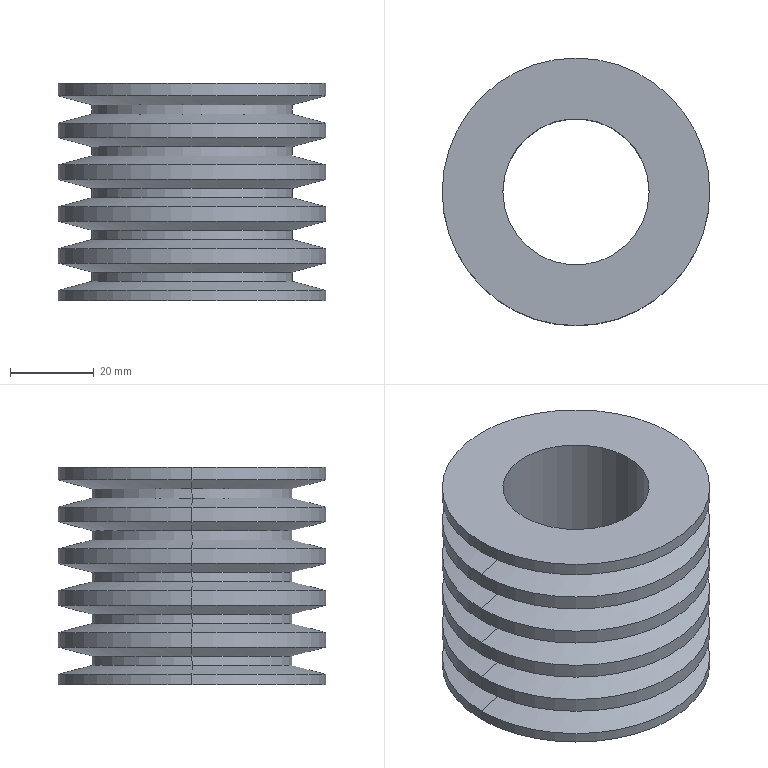Component | SolidWorks | SmallPulley-1 | 1 solid | 46 faces | box 64 x 64 x 52 mm | volume 85635 mm3 | cylinder 24 | cone 20 | plane 2 | commonest cylinder face diameters 64 x12 48 x10 35 x2
build123d program:
from build123d import *


with BuildPart() as part:
    # Sketch1 → Revolve1 (revolve)
    with BuildSketch(Plane(origin=(0, 0, 0), x_dir=(0, 0, -1), z_dir=(1, 0, 0)), mode=Mode.PRIVATE) as revolve1_sk:
        Polygon((49.535, 0), (52, 0), (52, -14.5), (0, -14.5), (0, 0), (3, 0), (5.144, -8), (7.391, -8), (9.535, 0), (13, 0), (15.144, -8), (17.391, -8), (19.535, 0), (23, 0), (25.144, -8), (27.391, -8), (29.535, 0), (33, 0), (35.144, -8), (37.391, -8), (39.535, 0), (43, 0), (45.144, -8), (47.391, -8), align=None)
    revolve(revolve1_sk.sketch.rotate(Axis((0, -32, 0), (0, 0, -1)), 90), axis=Axis((0, -32, 0), (0, 0, -1)))


solid = part.part

# Placed as in the assembly
solid = solid.moved(Location((549.733, 47.31, 121.5), (0, 0, 0)))